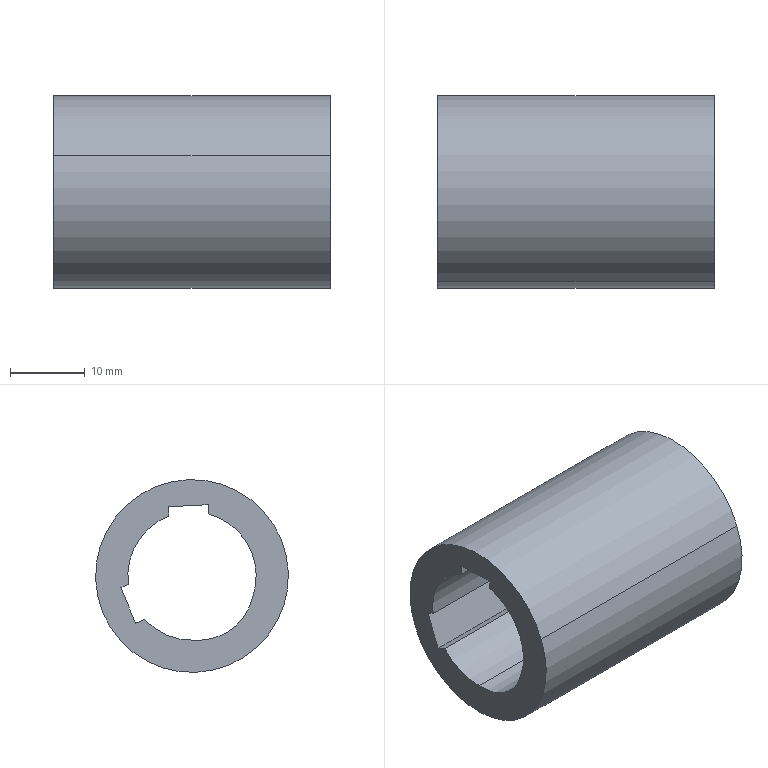Component | SolidWorks | CouplingSleeve-1 | 1 solid | 15 faces | box 37 x 25.76 x 25.76 mm | volume 10280 mm3 | plane 8 | cylinder 7 | commonest cylinder face diameters 17.16 x4 25.756 x2 15 x1
build123d program:
from build123d import *

# Parameters (mm, degrees)
SKETCH2_R               = 12.878
SKETCH2_R_2             = 8.58
BOSS_EXTRUDE1_DEPTH     = 37
CUT_EXTRUDE1_DEPTH      = 66.986
CUT_EXTRUDE1_DEPTH_BACK = 66.986
BOSS_EXTRUDE3_START     = -203.5
BOSS_EXTRUDE3_DEPTH     = 38


with BuildPart() as part:
    # Sketch2 → Boss-Extrude1 (new body)
    with BuildSketch(Plane(origin=(-166, 0, 0), x_dir=(0, 0, -1), z_dir=(1, 0, 0))):
        with Locations((-40.219, 0)):
            Circle(SKETCH2_R)
        with Locations((-40.219, 0)):
            Circle(SKETCH2_R_2, mode=Mode.SUBTRACT)
    extrude(amount=-BOSS_EXTRUDE1_DEPTH)

    # Sketch4 → Cut-Extrude1 (cut, two sides: drawn at the far end of the back side and taken through both)
    with BuildSketch(Plane(origin=(-166, 0, 0), x_dir=(0, 0, -1), z_dir=(1, 0, 0)).offset(-CUT_EXTRUDE1_DEPTH_BACK)):
        with BuildLine():
            Line((-46.528, -2.177), (-49.594, -2.177))
            Line((-49.594, -2.177), (-49.594, 3.001))
            Line((-49.594, 3.001), (-47.204, 3.001))
            ThreePointArc((-47.204, 3.001), (-32.458, 2.295), (-46.528, -2.177))
        make_face()
    extrude(amount=CUT_EXTRUDE1_DEPTH + CUT_EXTRUDE1_DEPTH_BACK, mode=Mode.SUBTRACT)


with BuildPart() as body_2:
    # Sketch3 → Boss-Extrude3 (new body)
    with BuildSketch(Plane(origin=(0, 0, 0), x_dir=(0, 0, -1), z_dir=(1, 0, 0)).offset(BOSS_EXTRUDE3_START)):
        Polygon((-35.481, -5.551), (-40.486, -7.293), (-39.632, -9.749), (-34.626, -8.006), align=None)
    extrude(amount=BOSS_EXTRUDE3_DEPTH)


with BuildPart() as part_1:
    add(part.part)

    # Combine1: cut body 2
    add(body_2.part, mode=Mode.SUBTRACT)


solid = part_1.part

# Placed as in the assembly
solid = solid.moved(Location((-83.5, 22.994, 15.228), (-112.249, 0, 0)))
STEP:
#1=COLOUR_RGB('',0.7922,0.8196,0.9333);
#2=FILL_AREA_STYLE_COLOUR('',#1);
#3=FILL_AREA_STYLE('',(#2));
#4=SURFACE_STYLE_FILL_AREA(#3);
#5=SURFACE_SIDE_STYLE('',(#4));
#6=SURFACE_STYLE_USAGE(.BOTH.,#5);
#7=PRESENTATION_STYLE_ASSIGNMENT((#6));
#8=CARTESIAN_POINT('',(-11.28,1.902,0.192));
#9=VERTEX_POINT('',#8);
#10=CARTESIAN_POINT('',(-11.28,2.84,-0.192));
#11=VERTEX_POINT('',#10);
#12=CARTESIAN_POINT('',(-11.28,2.371,-0.));
#13=DIRECTION('',(1.,0.,0.));
#14=DIRECTION('',(0.,-0.9255,0.3786));
#15=AXIS2_PLACEMENT_3D('',#12,#13,#14);
#16=CIRCLE('',#15,0.507);
#17=EDGE_CURVE('',#9,#11,#16,.T.);
#18=ORIENTED_EDGE('',*,*,#17,.T.);
#19=CARTESIAN_POINT('',(-9.823,2.84,-0.192));
#20=VERTEX_POINT('',#19);
#21=CARTESIAN_POINT('',(-11.28,2.84,-0.192));
#22=DIRECTION('',(1.,0.,0.));
#23=VECTOR('',#22,39.37);
#24=LINE('',#21,#23);
#25=EDGE_CURVE('',#11,#20,#24,.T.);
#26=ORIENTED_EDGE('',*,*,#25,.T.);
#27=CARTESIAN_POINT('',(-9.823,1.902,0.192));
#28=VERTEX_POINT('',#27);
#29=CARTESIAN_POINT('',(-9.823,2.371,-0.));
#30=DIRECTION('',(1.,0.,0.));
#31=DIRECTION('',(0.,-0.9255,0.3786));
#32=AXIS2_PLACEMENT_3D('',#29,#30,#31);
#33=CIRCLE('',#32,0.507);
#34=EDGE_CURVE('',#28,#20,#33,.T.);
#35=ORIENTED_EDGE('',*,*,#34,.F.);
#36=CARTESIAN_POINT('',(-11.28,1.902,0.192));
#37=DIRECTION('',(1.,0.,0.));
#38=VECTOR('',#37,39.37);
#39=LINE('',#36,#38);
#40=EDGE_CURVE('',#9,#28,#39,.T.);
#41=ORIENTED_EDGE('',*,*,#40,.F.);
#42=EDGE_LOOP('',(#18,#26,#35,#41));
#43=FACE_OUTER_BOUND('',#42,.T.);
#44=CARTESIAN_POINT('',(-11.28,2.371,-0.));
#45=DIRECTION('',(1.,0.,0.));
#46=DIRECTION('',(0.,-0.9255,0.3786));
#47=AXIS2_PLACEMENT_3D('',#44,#45,#46);
#48=CYLINDRICAL_SURFACE('',#47,0.507);
#49=ADVANCED_FACE('',(#43),#48,.T.);
#50=CARTESIAN_POINT('',(-11.28,2.058,0.1279));
#51=VERTEX_POINT('',#50);
#52=CARTESIAN_POINT('',(-11.28,2.052,-0.1116));
#53=VERTEX_POINT('',#52);
#54=CARTESIAN_POINT('',(-11.28,2.371,-0.));
#55=DIRECTION('',(1.,0.,0.));
#56=DIRECTION('',(0.,-0.9255,0.3786));
#57=AXIS2_PLACEMENT_3D('',#54,#55,#56);
#58=CIRCLE('',#57,0.3378);
#59=EDGE_CURVE('',#51,#53,#58,.T.);
#60=ORIENTED_EDGE('',*,*,#59,.F.);
#61=CARTESIAN_POINT('',(-9.823,2.058,0.1279));
#62=VERTEX_POINT('',#61);
#63=CARTESIAN_POINT('',(-11.28,2.058,0.1279));
#64=DIRECTION('',(1.,0.,0.));
#65=VECTOR('',#64,39.37);
#66=LINE('',#63,#65);
#67=EDGE_CURVE('',#51,#62,#66,.T.);
#68=ORIENTED_EDGE('',*,*,#67,.T.);
#69=CARTESIAN_POINT('',(-9.823,2.052,-0.1116));
#70=VERTEX_POINT('',#69);
#71=CARTESIAN_POINT('',(-9.823,2.371,-0.));
#72=DIRECTION('',(1.,0.,0.));
#73=DIRECTION('',(0.,-0.9255,0.3786));
#74=AXIS2_PLACEMENT_3D('',#71,#72,#73);
#75=CIRCLE('',#74,0.3378);
#76=EDGE_CURVE('',#62,#70,#75,.T.);
#77=ORIENTED_EDGE('',*,*,#76,.T.);
#78=CARTESIAN_POINT('',(-10.551,2.052,-0.1116));
#79=DIRECTION('',(-1.,0.,0.));
#80=VECTOR('',#79,39.37);
#81=LINE('',#78,#80);
#82=EDGE_CURVE('',#70,#53,#81,.T.);
#83=ORIENTED_EDGE('',*,*,#82,.T.);
#84=EDGE_LOOP('',(#60,#68,#77,#83));
#85=FACE_OUTER_BOUND('',#84,.T.);
#86=CARTESIAN_POINT('',(-11.28,2.371,-0.));
#87=DIRECTION('',(1.,0.,0.));
#88=DIRECTION('',(0.,-0.9255,0.3786));
#89=AXIS2_PLACEMENT_3D('',#86,#87,#88);
#90=CYLINDRICAL_SURFACE('',#89,0.3378);
#91=ADVANCED_FACE('',(#85),#90,.F.);
#92=ORIENTED_EDGE('',*,*,#17,.F.);
#93=CARTESIAN_POINT('',(-11.28,2.371,-0.));
#94=DIRECTION('',(1.,0.,0.));
#95=DIRECTION('',(0.,-0.9255,0.3786));
#96=AXIS2_PLACEMENT_3D('',#93,#94,#95);
#97=CIRCLE('',#96,0.507);
#98=EDGE_CURVE('',#11,#9,#97,.T.);
#99=ORIENTED_EDGE('',*,*,#98,.F.);
#100=EDGE_LOOP('',(#92,#99));
#101=FACE_OUTER_BOUND('',#100,.T.);
#102=CARTESIAN_POINT('',(-11.28,2.284,0.3264));
#103=VERTEX_POINT('',#102);
#104=CARTESIAN_POINT('',(-11.28,2.286,0.3751));
#105=VERTEX_POINT('',#104);
#106=CARTESIAN_POINT('',(-11.28,2.267,0.005565));
#107=DIRECTION('',(0.,0.05334,0.9986));
#108=VECTOR('',#107,39.37);
#109=LINE('',#106,#108);
#110=EDGE_CURVE('',#103,#105,#109,.T.);
#111=ORIENTED_EDGE('',*,*,#110,.F.);
#112=CARTESIAN_POINT('',(-11.28,2.371,-0.));
#113=DIRECTION('',(1.,0.,0.));
#114=DIRECTION('',(0.,-0.9255,0.3786));
#115=AXIS2_PLACEMENT_3D('',#112,#113,#114);
#116=CIRCLE('',#115,0.3378);
#117=EDGE_CURVE('',#103,#51,#116,.T.);
#118=ORIENTED_EDGE('',*,*,#117,.T.);
#119=ORIENTED_EDGE('',*,*,#59,.T.);
#120=CARTESIAN_POINT('',(-11.28,2.363,-0.3377));
#121=VERTEX_POINT('',#120);
#122=CARTESIAN_POINT('',(-11.28,2.339,-0.04337));
#123=DIRECTION('',(1.,0.,0.));
#124=DIRECTION('',(0.,-0.9255,0.3786));
#125=AXIS2_PLACEMENT_3D('',#122,#123,#124);
#126=CIRCLE('',#125,0.2953);
#127=EDGE_CURVE('',#53,#121,#126,.T.);
#128=ORIENTED_EDGE('',*,*,#127,.T.);
#129=CARTESIAN_POINT('',(-11.28,2.619,-0.2292));
#130=VERTEX_POINT('',#129);
#131=CARTESIAN_POINT('',(-11.28,2.371,-0.));
#132=DIRECTION('',(1.,0.,0.));
#133=DIRECTION('',(0.,-0.9255,0.3786));
#134=AXIS2_PLACEMENT_3D('',#131,#132,#133);
#135=CIRCLE('',#134,0.3378);
#136=EDGE_CURVE('',#121,#130,#135,.T.);
#137=ORIENTED_EDGE('',*,*,#136,.T.);
#138=CARTESIAN_POINT('',(-11.28,2.668,-0.2491));
#139=VERTEX_POINT('',#138);
#140=CARTESIAN_POINT('',(-11.28,2.668,-0.2491));
#141=DIRECTION('',(0.,0.9255,-0.3786));
#142=VECTOR('',#141,39.37);
#143=LINE('',#140,#142);
#144=EDGE_CURVE('',#130,#139,#143,.T.);
#145=ORIENTED_EDGE('',*,*,#144,.T.);
#146=CARTESIAN_POINT('',(-11.28,2.745,-0.06043));
#147=VERTEX_POINT('',#146);
#148=CARTESIAN_POINT('',(-11.28,2.745,-0.06043));
#149=DIRECTION('',(0.,0.3786,0.9255));
#150=VECTOR('',#149,39.37);
#151=LINE('',#148,#150);
#152=EDGE_CURVE('',#139,#147,#151,.T.);
#153=ORIENTED_EDGE('',*,*,#152,.T.);
#154=CARTESIAN_POINT('',(-11.28,2.706,-0.0444));
#155=VERTEX_POINT('',#154);
#156=CARTESIAN_POINT('',(-11.28,2.633,-0.01472));
#157=DIRECTION('',(0.,-0.9255,0.3786));
#158=VECTOR('',#157,39.37);
#159=LINE('',#156,#158);
#160=EDGE_CURVE('',#147,#155,#159,.T.);
#161=ORIENTED_EDGE('',*,*,#160,.T.);
#162=CARTESIAN_POINT('',(-11.28,2.492,0.3153));
#163=VERTEX_POINT('',#162);
#164=CARTESIAN_POINT('',(-11.28,2.371,-0.));
#165=DIRECTION('',(1.,0.,0.));
#166=DIRECTION('',(0.,-0.9255,0.3786));
#167=AXIS2_PLACEMENT_3D('',#164,#165,#166);
#168=CIRCLE('',#167,0.3378);
#169=EDGE_CURVE('',#155,#163,#168,.T.);
#170=ORIENTED_EDGE('',*,*,#169,.T.);
#171=CARTESIAN_POINT('',(-11.28,2.495,0.364));
#172=VERTEX_POINT('',#171);
#173=CARTESIAN_POINT('',(-11.28,2.475,-0.005564));
#174=DIRECTION('',(0.,-0.05333,-0.9986));
#175=VECTOR('',#174,39.37);
#176=LINE('',#173,#175);
#177=EDGE_CURVE('',#172,#163,#176,.T.);
#178=ORIENTED_EDGE('',*,*,#177,.F.);
#179=CARTESIAN_POINT('',(-11.28,2.391,0.3696));
#180=DIRECTION('',(0.,0.9986,-0.05333));
#181=VECTOR('',#180,39.37);
#182=LINE('',#179,#181);
#183=EDGE_CURVE('',#105,#172,#182,.T.);
#184=ORIENTED_EDGE('',*,*,#183,.F.);
#185=EDGE_LOOP('',(#111,#118,#119,#128,#137,#145,#153,#161,#170,#178,#184));
#186=FACE_BOUND('',#185,.T.);
#187=CARTESIAN_POINT('',(-11.28,2.371,-0.));
#188=DIRECTION('',(1.,0.,0.));
#189=DIRECTION('',(0.,-0.9255,0.3786));
#190=AXIS2_PLACEMENT_3D('',#187,#188,#189);
#191=PLANE('',#190);
#192=ADVANCED_FACE('',(#101,#186),#191,.F.);
#193=ORIENTED_EDGE('',*,*,#34,.T.);
#194=CARTESIAN_POINT('',(-9.823,2.371,-0.));
#195=DIRECTION('',(1.,0.,0.));
#196=DIRECTION('',(0.,-0.9255,0.3786));
#197=AXIS2_PLACEMENT_3D('',#194,#195,#196);
#198=CIRCLE('',#197,0.507);
#199=EDGE_CURVE('',#20,#28,#198,.T.);
#200=ORIENTED_EDGE('',*,*,#199,.T.);
#201=EDGE_LOOP('',(#193,#200));
#202=FACE_OUTER_BOUND('',#201,.T.);
#203=CARTESIAN_POINT('',(-9.823,2.284,0.3264));
#204=VERTEX_POINT('',#203);
#205=CARTESIAN_POINT('',(-9.823,2.371,-0.));
#206=DIRECTION('',(1.,0.,0.));
#207=DIRECTION('',(0.,-0.9255,0.3786));
#208=AXIS2_PLACEMENT_3D('',#205,#206,#207);
#209=CIRCLE('',#208,0.3378);
#210=EDGE_CURVE('',#204,#62,#209,.T.);
#211=ORIENTED_EDGE('',*,*,#210,.F.);
#212=CARTESIAN_POINT('',(-9.823,2.286,0.3751));
#213=VERTEX_POINT('',#212);
#214=CARTESIAN_POINT('',(-9.823,2.267,0.005565));
#215=DIRECTION('',(0.,0.05334,0.9986));
#216=VECTOR('',#215,39.37);
#217=LINE('',#214,#216);
#218=EDGE_CURVE('',#204,#213,#217,.T.);
#219=ORIENTED_EDGE('',*,*,#218,.T.);
#220=CARTESIAN_POINT('',(-9.823,2.495,0.364));
#221=VERTEX_POINT('',#220);
#222=CARTESIAN_POINT('',(-9.823,2.391,0.3696));
#223=DIRECTION('',(0.,0.9986,-0.05333));
#224=VECTOR('',#223,39.37);
#225=LINE('',#222,#224);
#226=EDGE_CURVE('',#213,#221,#225,.T.);
#227=ORIENTED_EDGE('',*,*,#226,.T.);
#228=CARTESIAN_POINT('',(-9.823,2.492,0.3153));
#229=VERTEX_POINT('',#228);
#230=CARTESIAN_POINT('',(-9.823,2.475,-0.005564));
#231=DIRECTION('',(0.,-0.05333,-0.9986));
#232=VECTOR('',#231,39.37);
#233=LINE('',#230,#232);
#234=EDGE_CURVE('',#221,#229,#233,.T.);
#235=ORIENTED_EDGE('',*,*,#234,.T.);
#236=CARTESIAN_POINT('',(-9.823,2.706,-0.0444));
#237=VERTEX_POINT('',#236);
#238=CARTESIAN_POINT('',(-9.823,2.371,-0.));
#239=DIRECTION('',(1.,0.,0.));
#240=DIRECTION('',(0.,-0.9255,0.3786));
#241=AXIS2_PLACEMENT_3D('',#238,#239,#240);
#242=CIRCLE('',#241,0.3378);
#243=EDGE_CURVE('',#237,#229,#242,.T.);
#244=ORIENTED_EDGE('',*,*,#243,.F.);
#245=CARTESIAN_POINT('',(-9.823,2.745,-0.06043));
#246=VERTEX_POINT('',#245);
#247=CARTESIAN_POINT('',(-9.823,2.403,0.07932));
#248=DIRECTION('',(0.,-0.9255,0.3786));
#249=VECTOR('',#248,39.37);
#250=LINE('',#247,#249);
#251=EDGE_CURVE('',#246,#237,#250,.T.);
#252=ORIENTED_EDGE('',*,*,#251,.F.);
#253=CARTESIAN_POINT('',(-9.823,2.668,-0.2491));
#254=VERTEX_POINT('',#253);
#255=CARTESIAN_POINT('',(-9.823,2.712,-0.1397));
#256=DIRECTION('',(0.,0.3786,0.9255));
#257=VECTOR('',#256,39.37);
#258=LINE('',#255,#257);
#259=EDGE_CURVE('',#254,#246,#258,.T.);
#260=ORIENTED_EDGE('',*,*,#259,.F.);
#261=CARTESIAN_POINT('',(-9.823,2.619,-0.2292));
#262=VERTEX_POINT('',#261);
#263=CARTESIAN_POINT('',(-9.823,2.326,-0.1093));
#264=DIRECTION('',(0.,0.9255,-0.3786));
#265=VECTOR('',#264,39.37);
#266=LINE('',#263,#265);
#267=EDGE_CURVE('',#262,#254,#266,.T.);
#268=ORIENTED_EDGE('',*,*,#267,.F.);
#269=CARTESIAN_POINT('',(-9.823,2.363,-0.3377));
#270=VERTEX_POINT('',#269);
#271=CARTESIAN_POINT('',(-9.823,2.371,-0.));
#272=DIRECTION('',(1.,0.,0.));
#273=DIRECTION('',(0.,-0.9255,0.3786));
#274=AXIS2_PLACEMENT_3D('',#271,#272,#273);
#275=CIRCLE('',#274,0.3378);
#276=EDGE_CURVE('',#270,#262,#275,.T.);
#277=ORIENTED_EDGE('',*,*,#276,.F.);
#278=CARTESIAN_POINT('',(-9.823,2.339,-0.04337));
#279=DIRECTION('',(1.,0.,0.));
#280=DIRECTION('',(0.,-0.9255,0.3786));
#281=AXIS2_PLACEMENT_3D('',#278,#279,#280);
#282=CIRCLE('',#281,0.2953);
#283=EDGE_CURVE('',#70,#270,#282,.T.);
#284=ORIENTED_EDGE('',*,*,#283,.F.);
#285=ORIENTED_EDGE('',*,*,#76,.F.);
#286=EDGE_LOOP('',(#211,#219,#227,#235,#244,#252,#260,#268,#277,#284,#285));
#287=FACE_BOUND('',#286,.T.);
#288=CARTESIAN_POINT('',(-9.823,2.371,-0.));
#289=DIRECTION('',(1.,0.,0.));
#290=DIRECTION('',(0.,-0.9255,0.3786));
#291=AXIS2_PLACEMENT_3D('',#288,#289,#290);
#292=PLANE('',#291);
#293=ADVANCED_FACE('',(#202,#287),#292,.T.);
#294=ORIENTED_EDGE('',*,*,#67,.F.);
#295=ORIENTED_EDGE('',*,*,#117,.F.);
#296=CARTESIAN_POINT('',(-11.28,2.284,0.3264));
#297=DIRECTION('',(-1.,0.,0.));
#298=VECTOR('',#297,39.37);
#299=LINE('',#296,#298);
#300=EDGE_CURVE('',#204,#103,#299,.T.);
#301=ORIENTED_EDGE('',*,*,#300,.F.);
#302=ORIENTED_EDGE('',*,*,#210,.T.);
#303=EDGE_LOOP('',(#294,#295,#301,#302));
#304=FACE_OUTER_BOUND('',#303,.T.);
#305=CARTESIAN_POINT('',(-11.28,2.371,-0.));
#306=DIRECTION('',(1.,0.,0.));
#307=DIRECTION('',(0.,-0.9255,0.3786));
#308=AXIS2_PLACEMENT_3D('',#305,#306,#307);
#309=CYLINDRICAL_SURFACE('',#308,0.3378);
#310=ADVANCED_FACE('',(#304),#309,.F.);
#311=CARTESIAN_POINT('',(-11.28,2.492,0.3153));
#312=DIRECTION('',(1.,0.,0.));
#313=VECTOR('',#312,39.37);
#314=LINE('',#311,#313);
#315=EDGE_CURVE('',#163,#229,#314,.T.);
#316=ORIENTED_EDGE('',*,*,#315,.F.);
#317=ORIENTED_EDGE('',*,*,#169,.F.);
#318=CARTESIAN_POINT('',(-11.28,2.706,-0.0444));
#319=DIRECTION('',(1.,0.,0.));
#320=VECTOR('',#319,39.37);
#321=LINE('',#318,#320);
#322=EDGE_CURVE('',#155,#237,#321,.T.);
#323=ORIENTED_EDGE('',*,*,#322,.T.);
#324=ORIENTED_EDGE('',*,*,#243,.T.);
#325=EDGE_LOOP('',(#316,#317,#323,#324));
#326=FACE_OUTER_BOUND('',#325,.T.);
#327=CARTESIAN_POINT('',(-11.28,2.371,-0.));
#328=DIRECTION('',(1.,0.,0.));
#329=DIRECTION('',(0.,-0.9255,0.3786));
#330=AXIS2_PLACEMENT_3D('',#327,#328,#329);
#331=CYLINDRICAL_SURFACE('',#330,0.3378);
#332=ADVANCED_FACE('',(#326),#331,.F.);
#333=ORIENTED_EDGE('',*,*,#136,.F.);
#334=CARTESIAN_POINT('',(-10.551,2.363,-0.3377));
#335=DIRECTION('',(1.,0.,0.));
#336=VECTOR('',#335,39.37);
#337=LINE('',#334,#336);
#338=EDGE_CURVE('',#121,#270,#337,.T.);
#339=ORIENTED_EDGE('',*,*,#338,.T.);
#340=ORIENTED_EDGE('',*,*,#276,.T.);
#341=CARTESIAN_POINT('',(-11.28,2.619,-0.2292));
#342=DIRECTION('',(-1.,0.,0.));
#343=VECTOR('',#342,39.37);
#344=LINE('',#341,#343);
#345=EDGE_CURVE('',#262,#130,#344,.T.);
#346=ORIENTED_EDGE('',*,*,#345,.T.);
#347=EDGE_LOOP('',(#333,#339,#340,#346));
#348=FACE_OUTER_BOUND('',#347,.T.);
#349=CARTESIAN_POINT('',(-11.28,2.371,-0.));
#350=DIRECTION('',(1.,0.,0.));
#351=DIRECTION('',(0.,-0.9255,0.3786));
#352=AXIS2_PLACEMENT_3D('',#349,#350,#351);
#353=CYLINDRICAL_SURFACE('',#352,0.3378);
#354=ADVANCED_FACE('',(#348),#353,.F.);
#355=ORIENTED_EDGE('',*,*,#25,.F.);
#356=ORIENTED_EDGE('',*,*,#98,.T.);
#357=ORIENTED_EDGE('',*,*,#40,.T.);
#358=ORIENTED_EDGE('',*,*,#199,.F.);
#359=EDGE_LOOP('',(#355,#356,#357,#358));
#360=FACE_OUTER_BOUND('',#359,.T.);
#361=CARTESIAN_POINT('',(-11.28,2.371,-0.));
#362=DIRECTION('',(1.,0.,0.));
#363=DIRECTION('',(0.,-0.9255,0.3786));
#364=AXIS2_PLACEMENT_3D('',#361,#362,#363);
#365=CYLINDRICAL_SURFACE('',#364,0.507);
#366=ADVANCED_FACE('',(#360),#365,.T.);
#367=ORIENTED_EDGE('',*,*,#251,.T.);
#368=ORIENTED_EDGE('',*,*,#322,.F.);
#369=ORIENTED_EDGE('',*,*,#160,.F.);
#370=CARTESIAN_POINT('',(-11.28,2.745,-0.06043));
#371=DIRECTION('',(1.,0.,0.));
#372=VECTOR('',#371,39.37);
#373=LINE('',#370,#372);
#374=EDGE_CURVE('',#147,#246,#373,.T.);
#375=ORIENTED_EDGE('',*,*,#374,.T.);
#376=EDGE_LOOP('',(#367,#368,#369,#375));
#377=FACE_OUTER_BOUND('',#376,.T.);
#378=CARTESIAN_POINT('',(-11.28,2.633,-0.01472));
#379=DIRECTION('',(0.,0.3786,0.9255));
#380=DIRECTION('',(0.,-0.9255,0.3786));
#381=AXIS2_PLACEMENT_3D('',#378,#379,#380);
#382=PLANE('',#381);
#383=ADVANCED_FACE('',(#377),#382,.F.);
#384=ORIENTED_EDGE('',*,*,#267,.T.);
#385=CARTESIAN_POINT('',(-11.28,2.668,-0.2491));
#386=DIRECTION('',(1.,0.,0.));
#387=VECTOR('',#386,39.37);
#388=LINE('',#385,#387);
#389=EDGE_CURVE('',#139,#254,#388,.T.);
#390=ORIENTED_EDGE('',*,*,#389,.F.);
#391=ORIENTED_EDGE('',*,*,#144,.F.);
#392=ORIENTED_EDGE('',*,*,#345,.F.);
#393=EDGE_LOOP('',(#384,#390,#391,#392));
#394=FACE_OUTER_BOUND('',#393,.T.);
#395=CARTESIAN_POINT('',(-11.28,2.668,-0.2491));
#396=DIRECTION('',(0.,-0.3786,-0.9255));
#397=DIRECTION('',(0.,0.9255,-0.3786));
#398=AXIS2_PLACEMENT_3D('',#395,#396,#397);
#399=PLANE('',#398);
#400=ADVANCED_FACE('',(#394),#399,.F.);
#401=ORIENTED_EDGE('',*,*,#259,.T.);
#402=ORIENTED_EDGE('',*,*,#374,.F.);
#403=ORIENTED_EDGE('',*,*,#152,.F.);
#404=ORIENTED_EDGE('',*,*,#389,.T.);
#405=EDGE_LOOP('',(#401,#402,#403,#404));
#406=FACE_OUTER_BOUND('',#405,.T.);
#407=CARTESIAN_POINT('',(-11.28,2.745,-0.06043));
#408=DIRECTION('',(0.,0.9255,-0.3786));
#409=DIRECTION('',(1.,0.,0.));
#410=AXIS2_PLACEMENT_3D('',#407,#408,#409);
#411=PLANE('',#410);
#412=ADVANCED_FACE('',(#406),#411,.F.);
#413=ORIENTED_EDGE('',*,*,#127,.F.);
#414=ORIENTED_EDGE('',*,*,#82,.F.);
#415=ORIENTED_EDGE('',*,*,#283,.T.);
#416=ORIENTED_EDGE('',*,*,#338,.F.);
#417=EDGE_LOOP('',(#413,#414,#415,#416));
#418=FACE_OUTER_BOUND('',#417,.T.);
#419=CARTESIAN_POINT('',(-11.28,2.339,-0.04337));
#420=DIRECTION('',(1.,0.,0.));
#421=DIRECTION('',(0.,-0.9255,0.3786));
#422=AXIS2_PLACEMENT_3D('',#419,#420,#421);
#423=CYLINDRICAL_SURFACE('',#422,0.2953);
#424=ADVANCED_FACE('',(#418),#423,.F.);
#425=ORIENTED_EDGE('',*,*,#183,.T.);
#426=CARTESIAN_POINT('',(-9.803,2.495,0.364));
#427=DIRECTION('',(-1.,0.,0.));
#428=VECTOR('',#427,39.37);
#429=LINE('',#426,#428);
#430=EDGE_CURVE('',#221,#172,#429,.T.);
#431=ORIENTED_EDGE('',*,*,#430,.F.);
#432=ORIENTED_EDGE('',*,*,#226,.F.);
#433=CARTESIAN_POINT('',(-9.803,2.286,0.3751));
#434=DIRECTION('',(-1.,0.,0.));
#435=VECTOR('',#434,39.37);
#436=LINE('',#433,#435);
#437=EDGE_CURVE('',#213,#105,#436,.T.);
#438=ORIENTED_EDGE('',*,*,#437,.T.);
#439=EDGE_LOOP('',(#425,#431,#432,#438));
#440=FACE_OUTER_BOUND('',#439,.T.);
#441=CARTESIAN_POINT('',(-9.803,2.495,0.364));
#442=DIRECTION('',(0.,-0.05333,-0.9986));
#443=DIRECTION('',(0.,0.9986,-0.05333));
#444=AXIS2_PLACEMENT_3D('',#441,#442,#443);
#445=PLANE('',#444);
#446=ADVANCED_FACE('',(#440),#445,.T.);
#447=ORIENTED_EDGE('',*,*,#110,.T.);
#448=ORIENTED_EDGE('',*,*,#437,.F.);
#449=ORIENTED_EDGE('',*,*,#218,.F.);
#450=ORIENTED_EDGE('',*,*,#300,.T.);
#451=EDGE_LOOP('',(#447,#448,#449,#450));
#452=FACE_OUTER_BOUND('',#451,.T.);
#453=CARTESIAN_POINT('',(-9.803,2.286,0.3751));
#454=DIRECTION('',(0.,0.9986,-0.05334));
#455=DIRECTION('',(0.,0.05334,0.9986));
#456=AXIS2_PLACEMENT_3D('',#453,#454,#455);
#457=PLANE('',#456);
#458=ADVANCED_FACE('',(#452),#457,.T.);
#459=ORIENTED_EDGE('',*,*,#177,.T.);
#460=ORIENTED_EDGE('',*,*,#315,.T.);
#461=ORIENTED_EDGE('',*,*,#234,.F.);
#462=ORIENTED_EDGE('',*,*,#430,.T.);
#463=EDGE_LOOP('',(#459,#460,#461,#462));
#464=FACE_OUTER_BOUND('',#463,.T.);
#465=CARTESIAN_POINT('',(-9.803,2.489,0.2618));
#466=DIRECTION('',(0.,-0.9986,0.05333));
#467=DIRECTION('',(0.,-0.05333,-0.9986));
#468=AXIS2_PLACEMENT_3D('',#465,#466,#467);
#469=PLANE('',#468);
#470=ADVANCED_FACE('',(#464),#469,.T.);
#471=CLOSED_SHELL('',(#49,#91,#192,#293,#310,#332,#354,#366,#383,#400,#412,#424,#446,#458,#470));
#472=MANIFOLD_SOLID_BREP('',#471);
#473=STYLED_ITEM('',(#7),#472);
#474=(LENGTH_UNIT()NAMED_UNIT(*)SI_UNIT($,.METRE.));
#475=LENGTH_MEASURE_WITH_UNIT(LENGTH_MEASURE(0.0254),#474);
#476=DIMENSIONAL_EXPONENTS(1.,0.,0.,0.,0.,0.,0.);
#477=(CONVERSION_BASED_UNIT('',#475)LENGTH_UNIT()NAMED_UNIT(#476));
#478=UNCERTAINTY_MEASURE_WITH_UNIT(LENGTH_MEASURE(0.00001),#477,'','');
#479=(NAMED_UNIT(*)PLANE_ANGLE_UNIT()SI_UNIT($,.RADIAN.));
#480=(NAMED_UNIT(*)SI_UNIT($,.STERADIAN.)SOLID_ANGLE_UNIT());
#481=(GEOMETRIC_REPRESENTATION_CONTEXT(3)GLOBAL_UNCERTAINTY_ASSIGNED_CONTEXT((#478))GLOBAL_UNIT_ASSIGNED_CONTEXT((#477,#479,#480))REPRESENTATION_CONTEXT('',''));
#482=MECHANICAL_DESIGN_GEOMETRIC_PRESENTATION_REPRESENTATION('',(#473),#481);
#483=CARTESIAN_POINT('',(0.,0.,0.));
#484=DIRECTION('',(0.,0.,1.));
#485=DIRECTION('',(1.,0.,0.));
#486=AXIS2_PLACEMENT_3D('',#483,#484,#485);
#487=(LENGTH_UNIT()NAMED_UNIT(*)SI_UNIT($,.METRE.));
#488=LENGTH_MEASURE_WITH_UNIT(LENGTH_MEASURE(0.0254),#487);
#489=DIMENSIONAL_EXPONENTS(1.,0.,0.,0.,0.,0.,0.);
#490=(CONVERSION_BASED_UNIT('',#488)LENGTH_UNIT()NAMED_UNIT(#489));
#491=UNCERTAINTY_MEASURE_WITH_UNIT(LENGTH_MEASURE(0.00001),#490,'','');
#492=(NAMED_UNIT(*)PLANE_ANGLE_UNIT()SI_UNIT($,.RADIAN.));
#493=(NAMED_UNIT(*)SI_UNIT($,.STERADIAN.)SOLID_ANGLE_UNIT());
#494=(GEOMETRIC_REPRESENTATION_CONTEXT(3)GLOBAL_UNCERTAINTY_ASSIGNED_CONTEXT((#491))GLOBAL_UNIT_ASSIGNED_CONTEXT((#490,#492,#493))REPRESENTATION_CONTEXT('',''));
#495=ADVANCED_BREP_SHAPE_REPRESENTATION('',(#472,#486),#494);
#496=PRESENTATION_LAYER_ASSIGNMENT('','',(#473));